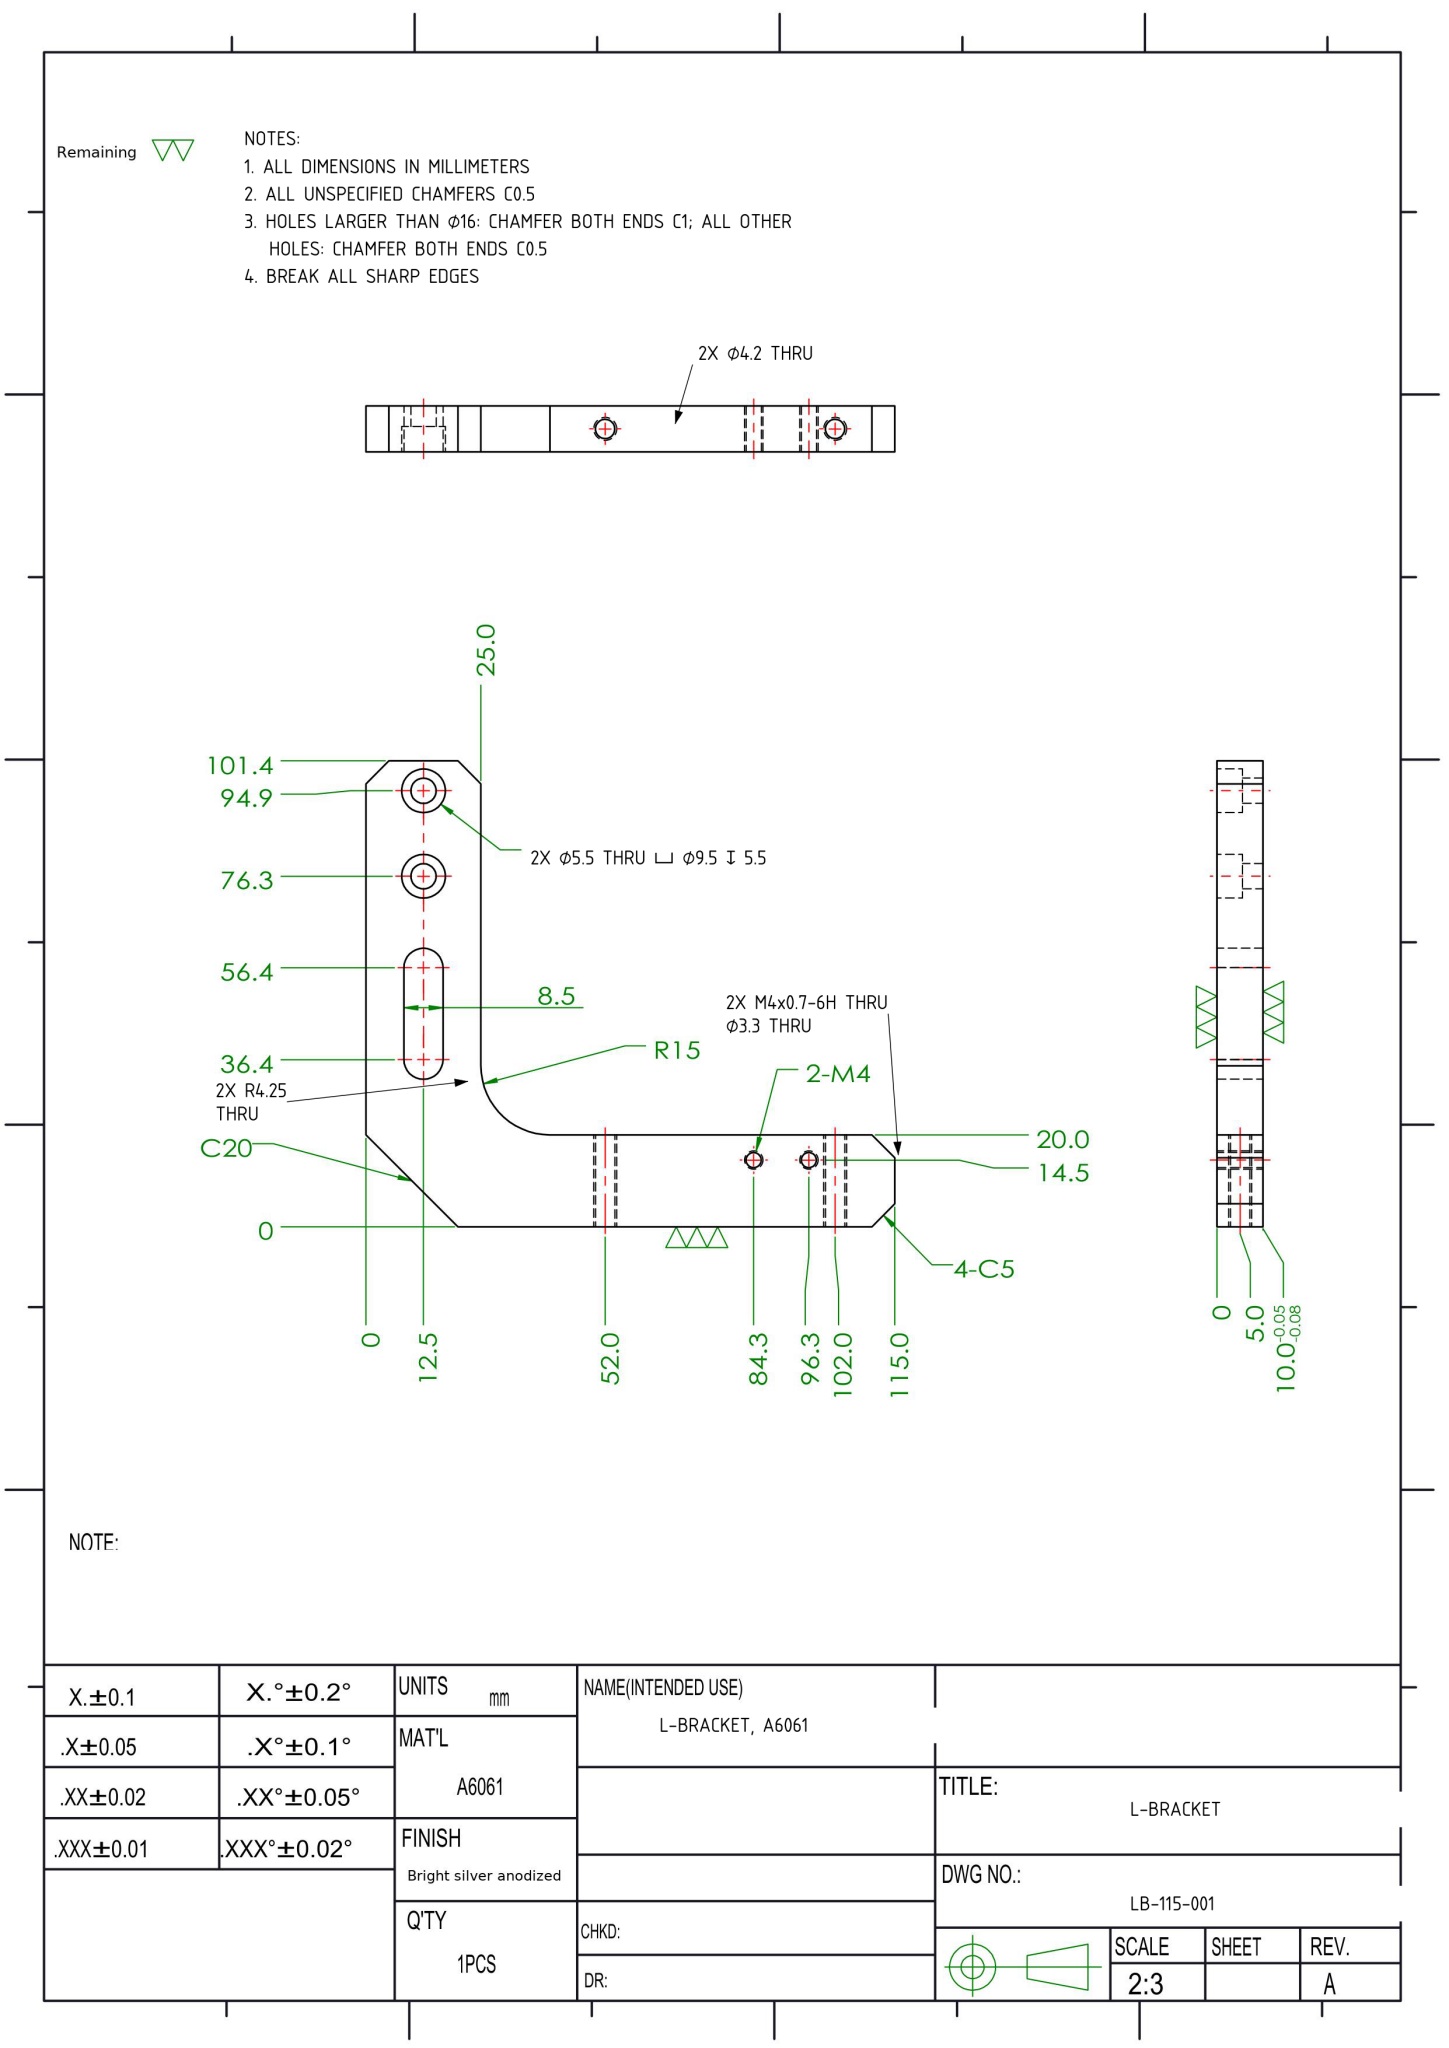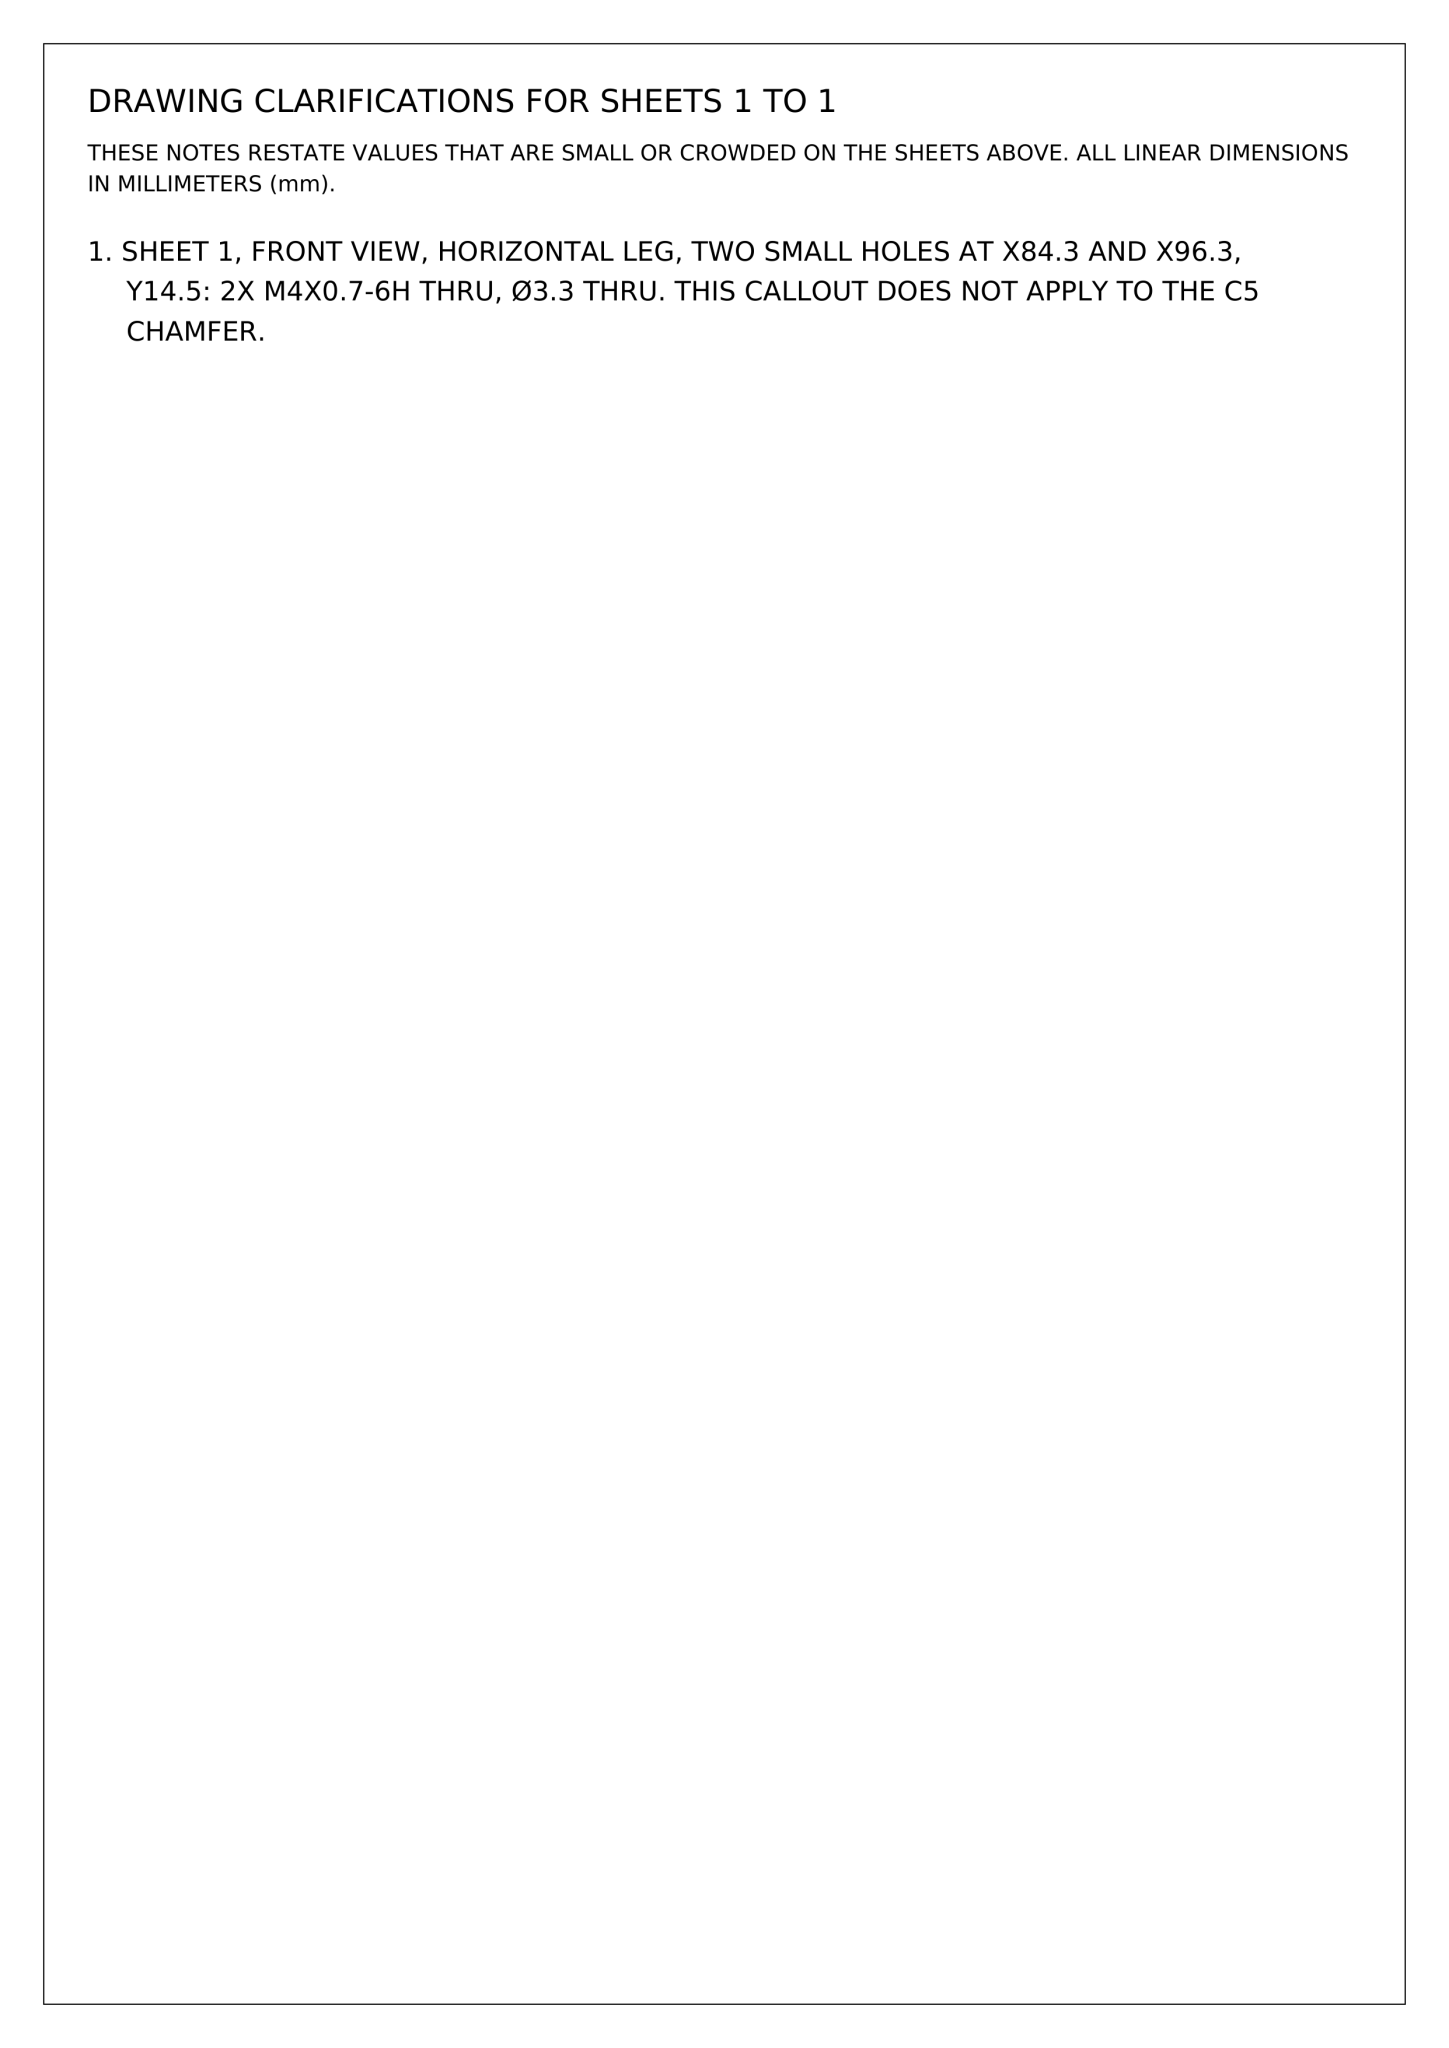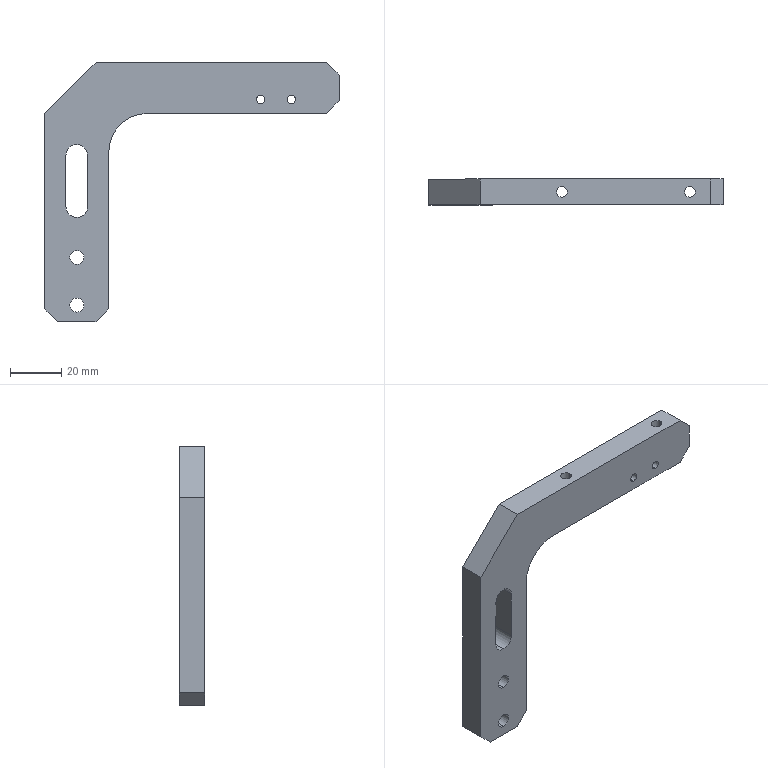Part | NX | mm | 1 solid | 37 faces | box 115 x 10 x 101.35 mm | volume 37334 mm3 | cylinder 20 | plane 17 | commonest cylinder face diameters 3.3 x4 4.2 x4 9.5 x4 5.5 x4 8.5 x3 30 x1